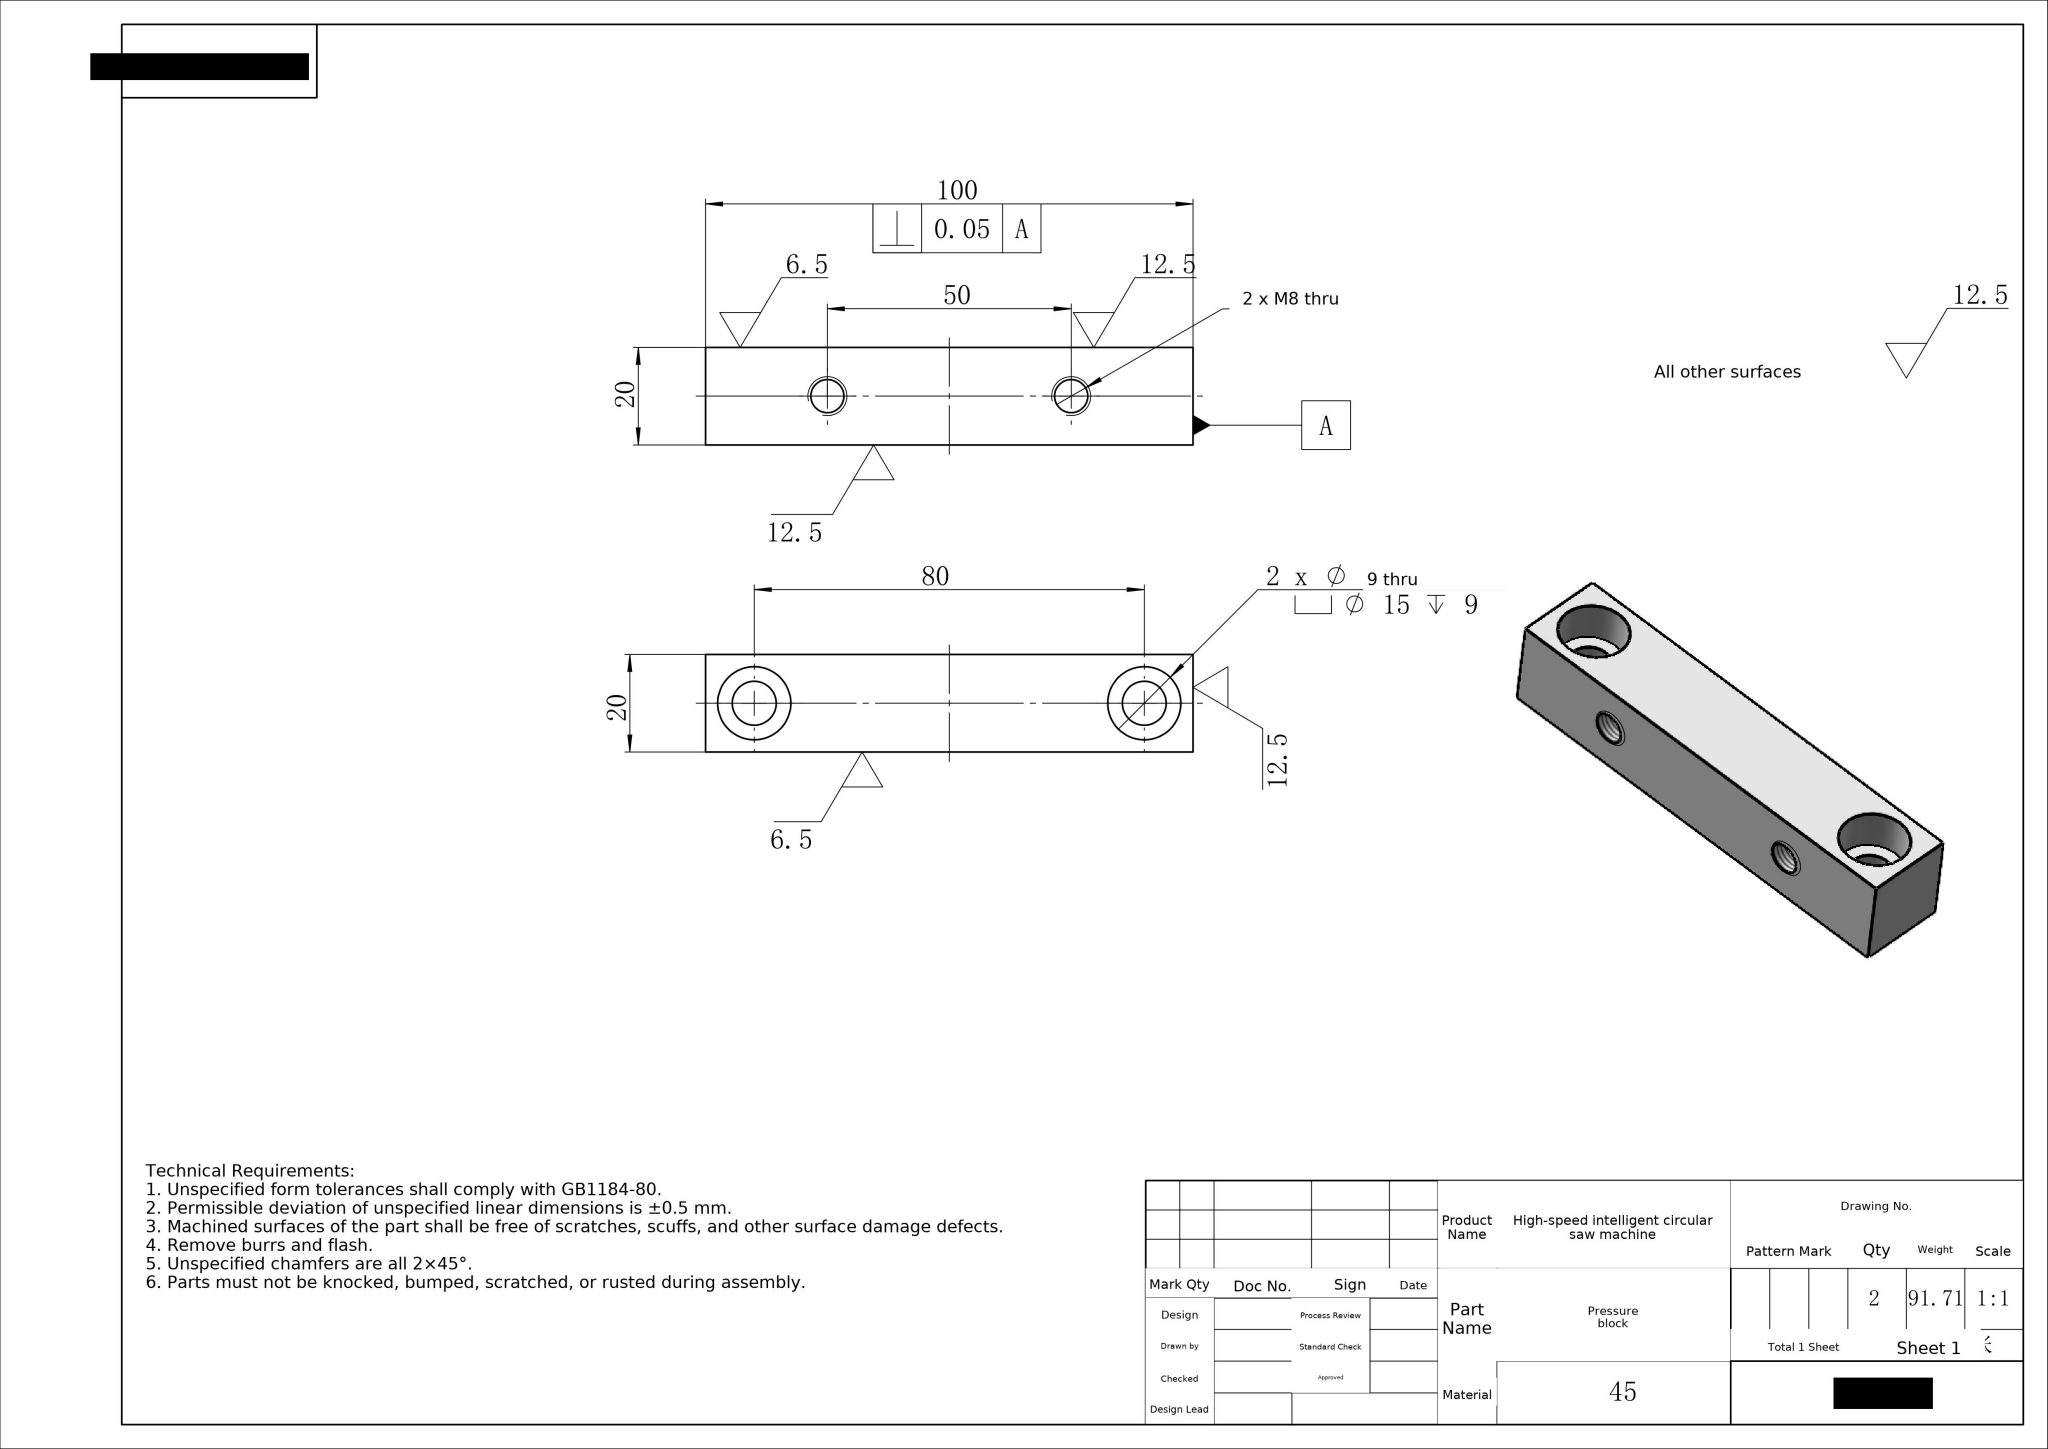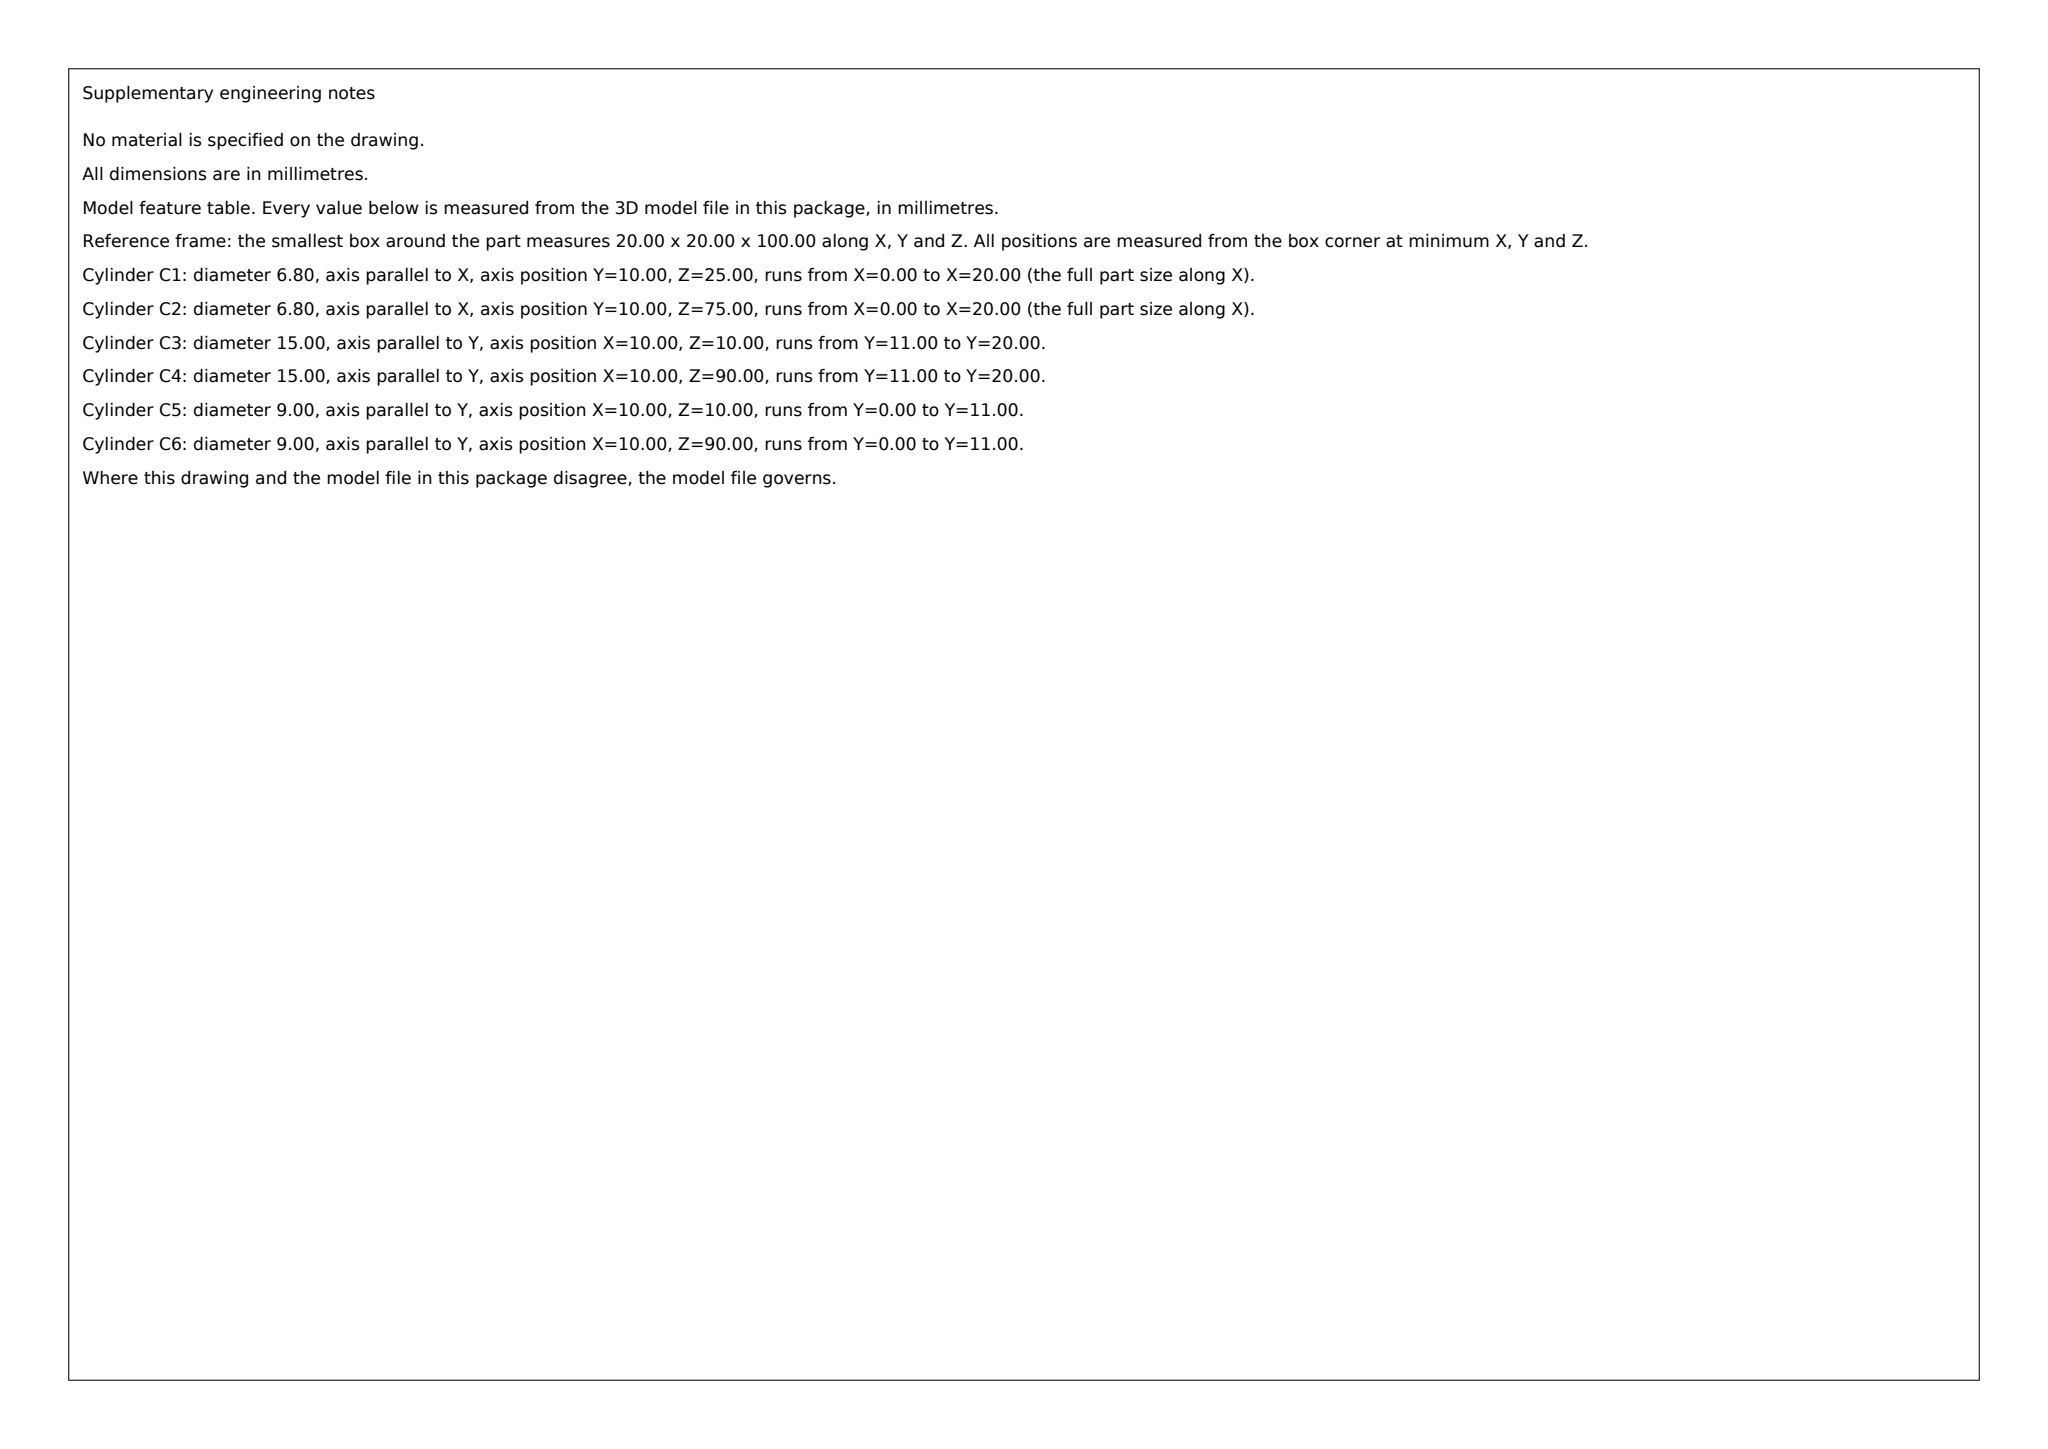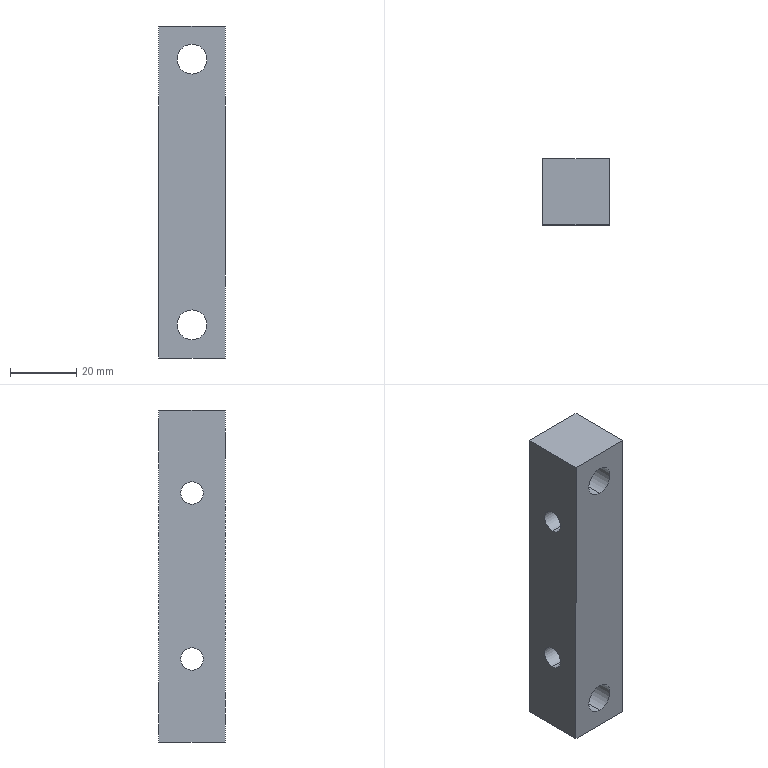Part | SolidWorks | mm | 1 solid | 20 faces | box 20 x 20 x 100 mm | volume 33967 mm3 | cylinder 12 | plane 8 | commonest cylinder face diameters 6.8 x4 15 x4 9 x4
build123d program:
from build123d import *

# Parameters (mm, degrees)
SKETCH2_W                                            = 20
SKETCH2_H                                            = 100
BOSS_EXTRUDE1_DEPTH                                  = 20
HOLE_SIZE_ACCORDING_TO_HEXAGON_SOCKET_HE_D           = 9
HOLE_SIZE_ACCORDING_TO_HEXAGON_SOCKET_HE_CBORE_D     = 15
HOLE_SIZE_ACCORDING_TO_HEXAGON_SOCKET_HE_CBORE_DEPTH = 9
M8_TAPPED_HOLE1_D                                    = 6.8


with BuildPart() as part:
    # Sketch2 → Boss-Extrude1 (new body)
    with BuildSketch(Plane(origin=(0, 0, 0), x_dir=(1, 0, 0), z_dir=(0, 1, 0))):
        Rectangle(SKETCH2_W, SKETCH2_H)
    extrude(amount=BOSS_EXTRUDE1_DEPTH)

    # Hole Size_According to_Hexagon Socket He (through all)
    with Locations(Plane(origin=(0, 20, -40), x_dir=(0, 0, 1), z_dir=(0, 1, 0))):
        with Locations((0, 0), (80, 0)):
            CounterBoreHole(HOLE_SIZE_ACCORDING_TO_HEXAGON_SOCKET_HE_D / 2, HOLE_SIZE_ACCORDING_TO_HEXAGON_SOCKET_HE_CBORE_D / 2, HOLE_SIZE_ACCORDING_TO_HEXAGON_SOCKET_HE_CBORE_DEPTH)

    # M8 Tapped Hole1 (through all)
    with Locations(Plane(origin=(-10, 10, -25), x_dir=(0, 0, -1), z_dir=(-1, 0, 0))):
        with Locations((0, 0), (-50, 0)):
            Hole(M8_TAPPED_HOLE1_D / 2)


solid = part.part
STEP:
#1=CARTESIAN_POINT('',(10.,10.,-28.4));
#2=VERTEX_POINT('',#1);
#3=CARTESIAN_POINT('',(10.,10.,-21.6));
#4=VERTEX_POINT('',#3);
#5=CARTESIAN_POINT('',(10.,10.,-25.));
#6=DIRECTION('',(-1.,0.,0.));
#7=DIRECTION('',(0.,0.,1.));
#8=AXIS2_PLACEMENT_3D('',#5,#6,#7);
#9=CIRCLE('',#8,3.4);
#10=EDGE_CURVE('',#2,#4,#9,.T.);
#11=ORIENTED_EDGE('',*,*,#10,.F.);
#12=CARTESIAN_POINT('',(-10.,10.,-28.4));
#13=VERTEX_POINT('',#12);
#14=CARTESIAN_POINT('',(-10.,10.,-28.4));
#15=DIRECTION('',(-1.,0.,0.));
#16=VECTOR('',#15,1000.);
#17=LINE('',#14,#16);
#18=EDGE_CURVE('',#2,#13,#17,.T.);
#19=ORIENTED_EDGE('',*,*,#18,.T.);
#20=CARTESIAN_POINT('',(-10.,10.,-21.6));
#21=VERTEX_POINT('',#20);
#22=CARTESIAN_POINT('',(-10.,10.,-25.));
#23=DIRECTION('',(-1.,0.,0.));
#24=DIRECTION('',(0.,0.,1.));
#25=AXIS2_PLACEMENT_3D('',#22,#23,#24);
#26=CIRCLE('',#25,3.4);
#27=EDGE_CURVE('',#13,#21,#26,.T.);
#28=ORIENTED_EDGE('',*,*,#27,.T.);
#29=CARTESIAN_POINT('',(-10.,10.,-21.6));
#30=DIRECTION('',(-1.,0.,0.));
#31=VECTOR('',#30,1000.);
#32=LINE('',#29,#31);
#33=EDGE_CURVE('',#4,#21,#32,.T.);
#34=ORIENTED_EDGE('',*,*,#33,.F.);
#35=EDGE_LOOP('',(#11,#19,#28,#34));
#36=FACE_OUTER_BOUND('',#35,.T.);
#37=CARTESIAN_POINT('',(-10.,10.,-25.));
#38=DIRECTION('',(-1.,0.,0.));
#39=DIRECTION('',(0.,0.,1.));
#40=AXIS2_PLACEMENT_3D('',#37,#38,#39);
#41=CYLINDRICAL_SURFACE('',#40,3.4);
#42=ADVANCED_FACE('',(#36),#41,.F.);
#43=CARTESIAN_POINT('',(10.,10.,21.6));
#44=VERTEX_POINT('',#43);
#45=CARTESIAN_POINT('',(10.,10.,28.4));
#46=VERTEX_POINT('',#45);
#47=CARTESIAN_POINT('',(10.,10.,25.));
#48=DIRECTION('',(-1.,0.,0.));
#49=DIRECTION('',(0.,0.,1.));
#50=AXIS2_PLACEMENT_3D('',#47,#48,#49);
#51=CIRCLE('',#50,3.4);
#52=EDGE_CURVE('',#44,#46,#51,.T.);
#53=ORIENTED_EDGE('',*,*,#52,.F.);
#54=CARTESIAN_POINT('',(-10.,10.,21.6));
#55=VERTEX_POINT('',#54);
#56=CARTESIAN_POINT('',(-10.,10.,21.6));
#57=DIRECTION('',(-1.,0.,0.));
#58=VECTOR('',#57,1000.);
#59=LINE('',#56,#58);
#60=EDGE_CURVE('',#44,#55,#59,.T.);
#61=ORIENTED_EDGE('',*,*,#60,.T.);
#62=CARTESIAN_POINT('',(-10.,10.,28.4));
#63=VERTEX_POINT('',#62);
#64=CARTESIAN_POINT('',(-10.,10.,25.));
#65=DIRECTION('',(-1.,0.,0.));
#66=DIRECTION('',(0.,0.,1.));
#67=AXIS2_PLACEMENT_3D('',#64,#65,#66);
#68=CIRCLE('',#67,3.4);
#69=EDGE_CURVE('',#55,#63,#68,.T.);
#70=ORIENTED_EDGE('',*,*,#69,.T.);
#71=CARTESIAN_POINT('',(-10.,10.,28.4));
#72=DIRECTION('',(-1.,0.,0.));
#73=VECTOR('',#72,1000.);
#74=LINE('',#71,#73);
#75=EDGE_CURVE('',#46,#63,#74,.T.);
#76=ORIENTED_EDGE('',*,*,#75,.F.);
#77=EDGE_LOOP('',(#53,#61,#70,#76));
#78=FACE_OUTER_BOUND('',#77,.T.);
#79=CARTESIAN_POINT('',(-10.,10.,25.));
#80=DIRECTION('',(-1.,0.,0.));
#81=DIRECTION('',(0.,0.,1.));
#82=AXIS2_PLACEMENT_3D('',#79,#80,#81);
#83=CYLINDRICAL_SURFACE('',#82,3.4);
#84=ADVANCED_FACE('',(#78),#83,.F.);
#85=CARTESIAN_POINT('',(0.,11.,-47.5));
#86=VERTEX_POINT('',#85);
#87=CARTESIAN_POINT('',(0.,11.,-32.5));
#88=VERTEX_POINT('',#87);
#89=CARTESIAN_POINT('',(0.,11.,-40.));
#90=DIRECTION('',(0.,1.,0.));
#91=DIRECTION('',(0.,0.,1.));
#92=AXIS2_PLACEMENT_3D('',#89,#90,#91);
#93=CIRCLE('',#92,7.5);
#94=EDGE_CURVE('',#86,#88,#93,.T.);
#95=ORIENTED_EDGE('',*,*,#94,.F.);
#96=CARTESIAN_POINT('',(0.,20.,-47.5));
#97=VERTEX_POINT('',#96);
#98=CARTESIAN_POINT('',(0.,20.,-47.5));
#99=DIRECTION('',(0.,1.,0.));
#100=VECTOR('',#99,1000.);
#101=LINE('',#98,#100);
#102=EDGE_CURVE('',#86,#97,#101,.T.);
#103=ORIENTED_EDGE('',*,*,#102,.T.);
#104=CARTESIAN_POINT('',(0.,20.,-32.5));
#105=VERTEX_POINT('',#104);
#106=CARTESIAN_POINT('',(0.,20.,-40.));
#107=DIRECTION('',(0.,1.,0.));
#108=DIRECTION('',(0.,0.,1.));
#109=AXIS2_PLACEMENT_3D('',#106,#107,#108);
#110=CIRCLE('',#109,7.5);
#111=EDGE_CURVE('',#97,#105,#110,.T.);
#112=ORIENTED_EDGE('',*,*,#111,.T.);
#113=CARTESIAN_POINT('',(0.,20.,-32.5));
#114=DIRECTION('',(0.,1.,0.));
#115=VECTOR('',#114,1000.);
#116=LINE('',#113,#115);
#117=EDGE_CURVE('',#88,#105,#116,.T.);
#118=ORIENTED_EDGE('',*,*,#117,.F.);
#119=EDGE_LOOP('',(#95,#103,#112,#118));
#120=FACE_OUTER_BOUND('',#119,.T.);
#121=CARTESIAN_POINT('',(0.,20.,-40.));
#122=DIRECTION('',(0.,1.,0.));
#123=DIRECTION('',(0.,0.,1.));
#124=AXIS2_PLACEMENT_3D('',#121,#122,#123);
#125=CYLINDRICAL_SURFACE('',#124,7.5);
#126=ADVANCED_FACE('',(#120),#125,.F.);
#127=CARTESIAN_POINT('',(0.,0.,-44.5));
#128=VERTEX_POINT('',#127);
#129=CARTESIAN_POINT('',(0.,0.,-35.5));
#130=VERTEX_POINT('',#129);
#131=CARTESIAN_POINT('',(0.,0.,-40.));
#132=DIRECTION('',(0.,1.,0.));
#133=DIRECTION('',(0.,0.,1.));
#134=AXIS2_PLACEMENT_3D('',#131,#132,#133);
#135=CIRCLE('',#134,4.5);
#136=EDGE_CURVE('',#128,#130,#135,.T.);
#137=ORIENTED_EDGE('',*,*,#136,.F.);
#138=CARTESIAN_POINT('',(0.,11.,-44.5));
#139=VERTEX_POINT('',#138);
#140=CARTESIAN_POINT('',(0.,20.,-44.5));
#141=DIRECTION('',(0.,1.,0.));
#142=VECTOR('',#141,1000.);
#143=LINE('',#140,#142);
#144=EDGE_CURVE('',#128,#139,#143,.T.);
#145=ORIENTED_EDGE('',*,*,#144,.T.);
#146=CARTESIAN_POINT('',(0.,11.,-35.5));
#147=VERTEX_POINT('',#146);
#148=CARTESIAN_POINT('',(0.,11.,-40.));
#149=DIRECTION('',(0.,1.,0.));
#150=DIRECTION('',(0.,0.,1.));
#151=AXIS2_PLACEMENT_3D('',#148,#149,#150);
#152=CIRCLE('',#151,4.5);
#153=EDGE_CURVE('',#139,#147,#152,.T.);
#154=ORIENTED_EDGE('',*,*,#153,.T.);
#155=CARTESIAN_POINT('',(0.,20.,-35.5));
#156=DIRECTION('',(0.,1.,0.));
#157=VECTOR('',#156,1000.);
#158=LINE('',#155,#157);
#159=EDGE_CURVE('',#130,#147,#158,.T.);
#160=ORIENTED_EDGE('',*,*,#159,.F.);
#161=EDGE_LOOP('',(#137,#145,#154,#160));
#162=FACE_OUTER_BOUND('',#161,.T.);
#163=CARTESIAN_POINT('',(0.,20.,-40.));
#164=DIRECTION('',(0.,1.,0.));
#165=DIRECTION('',(0.,0.,1.));
#166=AXIS2_PLACEMENT_3D('',#163,#164,#165);
#167=CYLINDRICAL_SURFACE('',#166,4.5);
#168=ADVANCED_FACE('',(#162),#167,.F.);
#169=CARTESIAN_POINT('',(0.,11.,32.5));
#170=VERTEX_POINT('',#169);
#171=CARTESIAN_POINT('',(0.,11.,47.5));
#172=VERTEX_POINT('',#171);
#173=CARTESIAN_POINT('',(0.,11.,40.));
#174=DIRECTION('',(0.,1.,0.));
#175=DIRECTION('',(0.,0.,1.));
#176=AXIS2_PLACEMENT_3D('',#173,#174,#175);
#177=CIRCLE('',#176,7.5);
#178=EDGE_CURVE('',#170,#172,#177,.T.);
#179=ORIENTED_EDGE('',*,*,#178,.F.);
#180=CARTESIAN_POINT('',(0.,20.,32.5));
#181=VERTEX_POINT('',#180);
#182=CARTESIAN_POINT('',(0.,20.,32.5));
#183=DIRECTION('',(0.,1.,0.));
#184=VECTOR('',#183,1000.);
#185=LINE('',#182,#184);
#186=EDGE_CURVE('',#170,#181,#185,.T.);
#187=ORIENTED_EDGE('',*,*,#186,.T.);
#188=CARTESIAN_POINT('',(0.,20.,47.5));
#189=VERTEX_POINT('',#188);
#190=CARTESIAN_POINT('',(0.,20.,40.));
#191=DIRECTION('',(0.,1.,0.));
#192=DIRECTION('',(0.,0.,1.));
#193=AXIS2_PLACEMENT_3D('',#190,#191,#192);
#194=CIRCLE('',#193,7.5);
#195=EDGE_CURVE('',#181,#189,#194,.T.);
#196=ORIENTED_EDGE('',*,*,#195,.T.);
#197=CARTESIAN_POINT('',(0.,20.,47.5));
#198=DIRECTION('',(0.,1.,0.));
#199=VECTOR('',#198,1000.);
#200=LINE('',#197,#199);
#201=EDGE_CURVE('',#172,#189,#200,.T.);
#202=ORIENTED_EDGE('',*,*,#201,.F.);
#203=EDGE_LOOP('',(#179,#187,#196,#202));
#204=FACE_OUTER_BOUND('',#203,.T.);
#205=CARTESIAN_POINT('',(0.,20.,40.));
#206=DIRECTION('',(0.,1.,0.));
#207=DIRECTION('',(0.,0.,1.));
#208=AXIS2_PLACEMENT_3D('',#205,#206,#207);
#209=CYLINDRICAL_SURFACE('',#208,7.5);
#210=ADVANCED_FACE('',(#204),#209,.F.);
#211=CARTESIAN_POINT('',(0.,0.,35.5));
#212=VERTEX_POINT('',#211);
#213=CARTESIAN_POINT('',(0.,0.,44.5));
#214=VERTEX_POINT('',#213);
#215=CARTESIAN_POINT('',(0.,0.,40.));
#216=DIRECTION('',(0.,1.,0.));
#217=DIRECTION('',(0.,0.,1.));
#218=AXIS2_PLACEMENT_3D('',#215,#216,#217);
#219=CIRCLE('',#218,4.5);
#220=EDGE_CURVE('',#212,#214,#219,.T.);
#221=ORIENTED_EDGE('',*,*,#220,.F.);
#222=CARTESIAN_POINT('',(0.,11.,35.5));
#223=VERTEX_POINT('',#222);
#224=CARTESIAN_POINT('',(0.,20.,35.5));
#225=DIRECTION('',(0.,1.,0.));
#226=VECTOR('',#225,1000.);
#227=LINE('',#224,#226);
#228=EDGE_CURVE('',#212,#223,#227,.T.);
#229=ORIENTED_EDGE('',*,*,#228,.T.);
#230=CARTESIAN_POINT('',(0.,11.,44.5));
#231=VERTEX_POINT('',#230);
#232=CARTESIAN_POINT('',(0.,11.,40.));
#233=DIRECTION('',(0.,1.,0.));
#234=DIRECTION('',(0.,0.,1.));
#235=AXIS2_PLACEMENT_3D('',#232,#233,#234);
#236=CIRCLE('',#235,4.5);
#237=EDGE_CURVE('',#223,#231,#236,.T.);
#238=ORIENTED_EDGE('',*,*,#237,.T.);
#239=CARTESIAN_POINT('',(0.,20.,44.5));
#240=DIRECTION('',(0.,1.,0.));
#241=VECTOR('',#240,1000.);
#242=LINE('',#239,#241);
#243=EDGE_CURVE('',#214,#231,#242,.T.);
#244=ORIENTED_EDGE('',*,*,#243,.F.);
#245=EDGE_LOOP('',(#221,#229,#238,#244));
#246=FACE_OUTER_BOUND('',#245,.T.);
#247=CARTESIAN_POINT('',(0.,20.,40.));
#248=DIRECTION('',(0.,1.,0.));
#249=DIRECTION('',(0.,0.,1.));
#250=AXIS2_PLACEMENT_3D('',#247,#248,#249);
#251=CYLINDRICAL_SURFACE('',#250,4.5);
#252=ADVANCED_FACE('',(#246),#251,.F.);
#253=CARTESIAN_POINT('',(10.,10.,-25.));
#254=DIRECTION('',(-1.,0.,0.));
#255=DIRECTION('',(0.,0.,1.));
#256=AXIS2_PLACEMENT_3D('',#253,#254,#255);
#257=CIRCLE('',#256,3.4);
#258=EDGE_CURVE('',#4,#2,#257,.T.);
#259=ORIENTED_EDGE('',*,*,#258,.T.);
#260=ORIENTED_EDGE('',*,*,#10,.T.);
#261=EDGE_LOOP('',(#259,#260));
#262=FACE_BOUND('',#261,.T.);
#263=CARTESIAN_POINT('',(10.,10.,25.));
#264=DIRECTION('',(-1.,0.,0.));
#265=DIRECTION('',(0.,0.,1.));
#266=AXIS2_PLACEMENT_3D('',#263,#264,#265);
#267=CIRCLE('',#266,3.4);
#268=EDGE_CURVE('',#46,#44,#267,.T.);
#269=ORIENTED_EDGE('',*,*,#268,.T.);
#270=ORIENTED_EDGE('',*,*,#52,.T.);
#271=EDGE_LOOP('',(#269,#270));
#272=FACE_BOUND('',#271,.T.);
#273=CARTESIAN_POINT('',(10.,0.,50.));
#274=VERTEX_POINT('',#273);
#275=CARTESIAN_POINT('',(10.,0.,-50.));
#276=VERTEX_POINT('',#275);
#277=CARTESIAN_POINT('',(10.,0.,-50.));
#278=DIRECTION('',(-0.,0.,-1.));
#279=VECTOR('',#278,1000.);
#280=LINE('',#277,#279);
#281=EDGE_CURVE('',#274,#276,#280,.T.);
#282=ORIENTED_EDGE('',*,*,#281,.T.);
#283=CARTESIAN_POINT('',(10.,20.,-50.));
#284=VERTEX_POINT('',#283);
#285=CARTESIAN_POINT('',(10.,20.,-50.));
#286=DIRECTION('',(0.,-1.,0.));
#287=VECTOR('',#286,1000.);
#288=LINE('',#285,#287);
#289=EDGE_CURVE('',#284,#276,#288,.T.);
#290=ORIENTED_EDGE('',*,*,#289,.F.);
#291=CARTESIAN_POINT('',(10.,20.,50.));
#292=VERTEX_POINT('',#291);
#293=CARTESIAN_POINT('',(10.,20.,-50.));
#294=DIRECTION('',(-0.,0.,-1.));
#295=VECTOR('',#294,1000.);
#296=LINE('',#293,#295);
#297=EDGE_CURVE('',#292,#284,#296,.T.);
#298=ORIENTED_EDGE('',*,*,#297,.F.);
#299=CARTESIAN_POINT('',(10.,20.,50.));
#300=DIRECTION('',(0.,-1.,0.));
#301=VECTOR('',#300,1000.);
#302=LINE('',#299,#301);
#303=EDGE_CURVE('',#292,#274,#302,.T.);
#304=ORIENTED_EDGE('',*,*,#303,.T.);
#305=EDGE_LOOP('',(#282,#290,#298,#304));
#306=FACE_OUTER_BOUND('',#305,.T.);
#307=CARTESIAN_POINT('',(10.,20.,-50.));
#308=DIRECTION('',(-1.,0.,0.));
#309=DIRECTION('',(0.,0.,1.));
#310=AXIS2_PLACEMENT_3D('',#307,#308,#309);
#311=PLANE('',#310);
#312=ADVANCED_FACE('',(#262,#272,#306),#311,.F.);
#313=CARTESIAN_POINT('',(-10.,0.,-50.));
#314=VERTEX_POINT('',#313);
#315=CARTESIAN_POINT('',(-10.,0.,-50.));
#316=DIRECTION('',(-1.,0.,0.));
#317=VECTOR('',#316,1000.);
#318=LINE('',#315,#317);
#319=EDGE_CURVE('',#276,#314,#318,.T.);
#320=ORIENTED_EDGE('',*,*,#319,.T.);
#321=CARTESIAN_POINT('',(-10.,20.,-50.));
#322=VERTEX_POINT('',#321);
#323=CARTESIAN_POINT('',(-10.,20.,-50.));
#324=DIRECTION('',(0.,-1.,0.));
#325=VECTOR('',#324,1000.);
#326=LINE('',#323,#325);
#327=EDGE_CURVE('',#322,#314,#326,.T.);
#328=ORIENTED_EDGE('',*,*,#327,.F.);
#329=CARTESIAN_POINT('',(-10.,20.,-50.));
#330=DIRECTION('',(-1.,0.,0.));
#331=VECTOR('',#330,1000.);
#332=LINE('',#329,#331);
#333=EDGE_CURVE('',#284,#322,#332,.T.);
#334=ORIENTED_EDGE('',*,*,#333,.F.);
#335=ORIENTED_EDGE('',*,*,#289,.T.);
#336=EDGE_LOOP('',(#320,#328,#334,#335));
#337=FACE_OUTER_BOUND('',#336,.T.);
#338=CARTESIAN_POINT('',(-10.,20.,-50.));
#339=DIRECTION('',(0.,0.,1.));
#340=DIRECTION('',(1.,0.,0.));
#341=AXIS2_PLACEMENT_3D('',#338,#339,#340);
#342=PLANE('',#341);
#343=ADVANCED_FACE('',(#337),#342,.F.);
#344=CARTESIAN_POINT('',(-10.,10.,-25.));
#345=DIRECTION('',(-1.,0.,0.));
#346=DIRECTION('',(0.,0.,1.));
#347=AXIS2_PLACEMENT_3D('',#344,#345,#346);
#348=CIRCLE('',#347,3.4);
#349=EDGE_CURVE('',#21,#13,#348,.T.);
#350=ORIENTED_EDGE('',*,*,#349,.F.);
#351=ORIENTED_EDGE('',*,*,#27,.F.);
#352=EDGE_LOOP('',(#350,#351));
#353=FACE_BOUND('',#352,.T.);
#354=CARTESIAN_POINT('',(-10.,10.,25.));
#355=DIRECTION('',(-1.,0.,0.));
#356=DIRECTION('',(0.,0.,1.));
#357=AXIS2_PLACEMENT_3D('',#354,#355,#356);
#358=CIRCLE('',#357,3.4);
#359=EDGE_CURVE('',#63,#55,#358,.T.);
#360=ORIENTED_EDGE('',*,*,#359,.F.);
#361=ORIENTED_EDGE('',*,*,#69,.F.);
#362=EDGE_LOOP('',(#360,#361));
#363=FACE_BOUND('',#362,.T.);
#364=CARTESIAN_POINT('',(-10.,0.,50.));
#365=VERTEX_POINT('',#364);
#366=CARTESIAN_POINT('',(-10.,0.,-50.));
#367=DIRECTION('',(0.,0.,1.));
#368=VECTOR('',#367,1000.);
#369=LINE('',#366,#368);
#370=EDGE_CURVE('',#314,#365,#369,.T.);
#371=ORIENTED_EDGE('',*,*,#370,.T.);
#372=CARTESIAN_POINT('',(-10.,20.,50.));
#373=VERTEX_POINT('',#372);
#374=CARTESIAN_POINT('',(-10.,20.,50.));
#375=DIRECTION('',(0.,-1.,0.));
#376=VECTOR('',#375,1000.);
#377=LINE('',#374,#376);
#378=EDGE_CURVE('',#373,#365,#377,.T.);
#379=ORIENTED_EDGE('',*,*,#378,.F.);
#380=CARTESIAN_POINT('',(-10.,20.,-50.));
#381=DIRECTION('',(0.,0.,1.));
#382=VECTOR('',#381,1000.);
#383=LINE('',#380,#382);
#384=EDGE_CURVE('',#322,#373,#383,.T.);
#385=ORIENTED_EDGE('',*,*,#384,.F.);
#386=ORIENTED_EDGE('',*,*,#327,.T.);
#387=EDGE_LOOP('',(#371,#379,#385,#386));
#388=FACE_OUTER_BOUND('',#387,.T.);
#389=CARTESIAN_POINT('',(-10.,20.,-50.));
#390=DIRECTION('',(1.,0.,-0.));
#391=DIRECTION('',(-0.,0.,-1.));
#392=AXIS2_PLACEMENT_3D('',#389,#390,#391);
#393=PLANE('',#392);
#394=ADVANCED_FACE('',(#353,#363,#388),#393,.F.);
#395=CARTESIAN_POINT('',(-10.,0.,50.));
#396=DIRECTION('',(1.,0.,0.));
#397=VECTOR('',#396,1000.);
#398=LINE('',#395,#397);
#399=EDGE_CURVE('',#365,#274,#398,.T.);
#400=ORIENTED_EDGE('',*,*,#399,.T.);
#401=ORIENTED_EDGE('',*,*,#303,.F.);
#402=CARTESIAN_POINT('',(-10.,20.,50.));
#403=DIRECTION('',(1.,0.,0.));
#404=VECTOR('',#403,1000.);
#405=LINE('',#402,#404);
#406=EDGE_CURVE('',#373,#292,#405,.T.);
#407=ORIENTED_EDGE('',*,*,#406,.F.);
#408=ORIENTED_EDGE('',*,*,#378,.T.);
#409=EDGE_LOOP('',(#400,#401,#407,#408));
#410=FACE_OUTER_BOUND('',#409,.T.);
#411=CARTESIAN_POINT('',(-10.,20.,50.));
#412=DIRECTION('',(0.,0.,-1.));
#413=DIRECTION('',(-1.,0.,0.));
#414=AXIS2_PLACEMENT_3D('',#411,#412,#413);
#415=PLANE('',#414);
#416=ADVANCED_FACE('',(#410),#415,.F.);
#417=CARTESIAN_POINT('',(0.,20.,-40.));
#418=DIRECTION('',(0.,1.,0.));
#419=DIRECTION('',(0.,0.,1.));
#420=AXIS2_PLACEMENT_3D('',#417,#418,#419);
#421=CIRCLE('',#420,7.5);
#422=EDGE_CURVE('',#105,#97,#421,.T.);
#423=ORIENTED_EDGE('',*,*,#422,.F.);
#424=ORIENTED_EDGE('',*,*,#111,.F.);
#425=EDGE_LOOP('',(#423,#424));
#426=FACE_BOUND('',#425,.T.);
#427=CARTESIAN_POINT('',(0.,20.,40.));
#428=DIRECTION('',(0.,1.,0.));
#429=DIRECTION('',(0.,0.,1.));
#430=AXIS2_PLACEMENT_3D('',#427,#428,#429);
#431=CIRCLE('',#430,7.5);
#432=EDGE_CURVE('',#189,#181,#431,.T.);
#433=ORIENTED_EDGE('',*,*,#432,.F.);
#434=ORIENTED_EDGE('',*,*,#195,.F.);
#435=EDGE_LOOP('',(#433,#434));
#436=FACE_BOUND('',#435,.T.);
#437=ORIENTED_EDGE('',*,*,#297,.T.);
#438=ORIENTED_EDGE('',*,*,#333,.T.);
#439=ORIENTED_EDGE('',*,*,#384,.T.);
#440=ORIENTED_EDGE('',*,*,#406,.T.);
#441=EDGE_LOOP('',(#437,#438,#439,#440));
#442=FACE_OUTER_BOUND('',#441,.T.);
#443=CARTESIAN_POINT('',(0.,20.,0.));
#444=DIRECTION('',(0.,1.,0.));
#445=DIRECTION('',(0.,0.,1.));
#446=AXIS2_PLACEMENT_3D('',#443,#444,#445);
#447=PLANE('',#446);
#448=ADVANCED_FACE('',(#426,#436,#442),#447,.T.);
#449=CARTESIAN_POINT('',(0.,0.,-40.));
#450=DIRECTION('',(0.,1.,0.));
#451=DIRECTION('',(0.,0.,1.));
#452=AXIS2_PLACEMENT_3D('',#449,#450,#451);
#453=CIRCLE('',#452,4.5);
#454=EDGE_CURVE('',#130,#128,#453,.T.);
#455=ORIENTED_EDGE('',*,*,#454,.T.);
#456=ORIENTED_EDGE('',*,*,#136,.T.);
#457=EDGE_LOOP('',(#455,#456));
#458=FACE_BOUND('',#457,.T.);
#459=CARTESIAN_POINT('',(0.,0.,40.));
#460=DIRECTION('',(0.,1.,0.));
#461=DIRECTION('',(0.,0.,1.));
#462=AXIS2_PLACEMENT_3D('',#459,#460,#461);
#463=CIRCLE('',#462,4.5);
#464=EDGE_CURVE('',#214,#212,#463,.T.);
#465=ORIENTED_EDGE('',*,*,#464,.T.);
#466=ORIENTED_EDGE('',*,*,#220,.T.);
#467=EDGE_LOOP('',(#465,#466));
#468=FACE_BOUND('',#467,.T.);
#469=ORIENTED_EDGE('',*,*,#281,.F.);
#470=ORIENTED_EDGE('',*,*,#399,.F.);
#471=ORIENTED_EDGE('',*,*,#370,.F.);
#472=ORIENTED_EDGE('',*,*,#319,.F.);
#473=EDGE_LOOP('',(#469,#470,#471,#472));
#474=FACE_OUTER_BOUND('',#473,.T.);
#475=CARTESIAN_POINT('',(0.,0.,0.));
#476=DIRECTION('',(0.,1.,0.));
#477=DIRECTION('',(0.,0.,1.));
#478=AXIS2_PLACEMENT_3D('',#475,#476,#477);
#479=PLANE('',#478);
#480=ADVANCED_FACE('',(#458,#468,#474),#479,.F.);
#481=ORIENTED_EDGE('',*,*,#228,.F.);
#482=ORIENTED_EDGE('',*,*,#464,.F.);
#483=ORIENTED_EDGE('',*,*,#243,.T.);
#484=CARTESIAN_POINT('',(0.,11.,40.));
#485=DIRECTION('',(0.,1.,0.));
#486=DIRECTION('',(0.,0.,1.));
#487=AXIS2_PLACEMENT_3D('',#484,#485,#486);
#488=CIRCLE('',#487,4.5);
#489=EDGE_CURVE('',#231,#223,#488,.T.);
#490=ORIENTED_EDGE('',*,*,#489,.T.);
#491=EDGE_LOOP('',(#481,#482,#483,#490));
#492=FACE_OUTER_BOUND('',#491,.T.);
#493=CARTESIAN_POINT('',(0.,20.,40.));
#494=DIRECTION('',(0.,1.,0.));
#495=DIRECTION('',(0.,0.,1.));
#496=AXIS2_PLACEMENT_3D('',#493,#494,#495);
#497=CYLINDRICAL_SURFACE('',#496,4.5);
#498=ADVANCED_FACE('',(#492),#497,.F.);
#499=ORIENTED_EDGE('',*,*,#489,.F.);
#500=ORIENTED_EDGE('',*,*,#237,.F.);
#501=EDGE_LOOP('',(#499,#500));
#502=FACE_BOUND('',#501,.T.);
#503=CARTESIAN_POINT('',(0.,11.,40.));
#504=DIRECTION('',(0.,1.,0.));
#505=DIRECTION('',(0.,0.,1.));
#506=AXIS2_PLACEMENT_3D('',#503,#504,#505);
#507=CIRCLE('',#506,7.5);
#508=EDGE_CURVE('',#172,#170,#507,.T.);
#509=ORIENTED_EDGE('',*,*,#508,.T.);
#510=ORIENTED_EDGE('',*,*,#178,.T.);
#511=EDGE_LOOP('',(#509,#510));
#512=FACE_OUTER_BOUND('',#511,.T.);
#513=CARTESIAN_POINT('',(4.5,11.,40.));
#514=DIRECTION('',(0.,-1.,0.));
#515=DIRECTION('',(0.,0.,-1.));
#516=AXIS2_PLACEMENT_3D('',#513,#514,#515);
#517=PLANE('',#516);
#518=ADVANCED_FACE('',(#502,#512),#517,.F.);
#519=ORIENTED_EDGE('',*,*,#186,.F.);
#520=ORIENTED_EDGE('',*,*,#508,.F.);
#521=ORIENTED_EDGE('',*,*,#201,.T.);
#522=ORIENTED_EDGE('',*,*,#432,.T.);
#523=EDGE_LOOP('',(#519,#520,#521,#522));
#524=FACE_OUTER_BOUND('',#523,.T.);
#525=CARTESIAN_POINT('',(0.,20.,40.));
#526=DIRECTION('',(0.,1.,0.));
#527=DIRECTION('',(0.,0.,1.));
#528=AXIS2_PLACEMENT_3D('',#525,#526,#527);
#529=CYLINDRICAL_SURFACE('',#528,7.5);
#530=ADVANCED_FACE('',(#524),#529,.F.);
#531=ORIENTED_EDGE('',*,*,#144,.F.);
#532=ORIENTED_EDGE('',*,*,#454,.F.);
#533=ORIENTED_EDGE('',*,*,#159,.T.);
#534=CARTESIAN_POINT('',(0.,11.,-40.));
#535=DIRECTION('',(0.,1.,0.));
#536=DIRECTION('',(0.,0.,1.));
#537=AXIS2_PLACEMENT_3D('',#534,#535,#536);
#538=CIRCLE('',#537,4.5);
#539=EDGE_CURVE('',#147,#139,#538,.T.);
#540=ORIENTED_EDGE('',*,*,#539,.T.);
#541=EDGE_LOOP('',(#531,#532,#533,#540));
#542=FACE_OUTER_BOUND('',#541,.T.);
#543=CARTESIAN_POINT('',(0.,20.,-40.));
#544=DIRECTION('',(0.,1.,0.));
#545=DIRECTION('',(0.,0.,1.));
#546=AXIS2_PLACEMENT_3D('',#543,#544,#545);
#547=CYLINDRICAL_SURFACE('',#546,4.5);
#548=ADVANCED_FACE('',(#542),#547,.F.);
#549=ORIENTED_EDGE('',*,*,#539,.F.);
#550=ORIENTED_EDGE('',*,*,#153,.F.);
#551=EDGE_LOOP('',(#549,#550));
#552=FACE_BOUND('',#551,.T.);
#553=CARTESIAN_POINT('',(0.,11.,-40.));
#554=DIRECTION('',(0.,1.,0.));
#555=DIRECTION('',(0.,0.,1.));
#556=AXIS2_PLACEMENT_3D('',#553,#554,#555);
#557=CIRCLE('',#556,7.5);
#558=EDGE_CURVE('',#88,#86,#557,.T.);
#559=ORIENTED_EDGE('',*,*,#558,.T.);
#560=ORIENTED_EDGE('',*,*,#94,.T.);
#561=EDGE_LOOP('',(#559,#560));
#562=FACE_OUTER_BOUND('',#561,.T.);
#563=CARTESIAN_POINT('',(4.5,11.,-40.));
#564=DIRECTION('',(0.,-1.,0.));
#565=DIRECTION('',(0.,0.,-1.));
#566=AXIS2_PLACEMENT_3D('',#563,#564,#565);
#567=PLANE('',#566);
#568=ADVANCED_FACE('',(#552,#562),#567,.F.);
#569=ORIENTED_EDGE('',*,*,#102,.F.);
#570=ORIENTED_EDGE('',*,*,#558,.F.);
#571=ORIENTED_EDGE('',*,*,#117,.T.);
#572=ORIENTED_EDGE('',*,*,#422,.T.);
#573=EDGE_LOOP('',(#569,#570,#571,#572));
#574=FACE_OUTER_BOUND('',#573,.T.);
#575=CARTESIAN_POINT('',(0.,20.,-40.));
#576=DIRECTION('',(0.,1.,0.));
#577=DIRECTION('',(0.,0.,1.));
#578=AXIS2_PLACEMENT_3D('',#575,#576,#577);
#579=CYLINDRICAL_SURFACE('',#578,7.5);
#580=ADVANCED_FACE('',(#574),#579,.F.);
#581=ORIENTED_EDGE('',*,*,#60,.F.);
#582=ORIENTED_EDGE('',*,*,#268,.F.);
#583=ORIENTED_EDGE('',*,*,#75,.T.);
#584=ORIENTED_EDGE('',*,*,#359,.T.);
#585=EDGE_LOOP('',(#581,#582,#583,#584));
#586=FACE_OUTER_BOUND('',#585,.T.);
#587=CARTESIAN_POINT('',(-10.,10.,25.));
#588=DIRECTION('',(-1.,0.,0.));
#589=DIRECTION('',(0.,0.,1.));
#590=AXIS2_PLACEMENT_3D('',#587,#588,#589);
#591=CYLINDRICAL_SURFACE('',#590,3.4);
#592=ADVANCED_FACE('',(#586),#591,.F.);
#593=ORIENTED_EDGE('',*,*,#18,.F.);
#594=ORIENTED_EDGE('',*,*,#258,.F.);
#595=ORIENTED_EDGE('',*,*,#33,.T.);
#596=ORIENTED_EDGE('',*,*,#349,.T.);
#597=EDGE_LOOP('',(#593,#594,#595,#596));
#598=FACE_OUTER_BOUND('',#597,.T.);
#599=CARTESIAN_POINT('',(-10.,10.,-25.));
#600=DIRECTION('',(-1.,0.,0.));
#601=DIRECTION('',(0.,0.,1.));
#602=AXIS2_PLACEMENT_3D('',#599,#600,#601);
#603=CYLINDRICAL_SURFACE('',#602,3.4);
#604=ADVANCED_FACE('',(#598),#603,.F.);
#605=CLOSED_SHELL('',(#42,#84,#126,#168,#210,#252,#312,#343,#394,#416,#448,#480,#498,#518,#530,#548,#568,#580,#592,#604));
#606=MANIFOLD_SOLID_BREP('',#605);
#607=CARTESIAN_POINT('',(0.,0.,0.));
#608=DIRECTION('',(0.,0.,1.));
#609=DIRECTION('',(1.,0.,0.));
#610=AXIS2_PLACEMENT_3D('',#607,#608,#609);
#611=(LENGTH_UNIT()NAMED_UNIT(*)SI_UNIT(.MILLI.,.METRE.));
#612=UNCERTAINTY_MEASURE_WITH_UNIT(LENGTH_MEASURE(0.00001),#611,'','');
#613=(NAMED_UNIT(*)PLANE_ANGLE_UNIT()SI_UNIT($,.RADIAN.));
#614=(NAMED_UNIT(*)SI_UNIT($,.STERADIAN.)SOLID_ANGLE_UNIT());
#615=(GEOMETRIC_REPRESENTATION_CONTEXT(3)GLOBAL_UNCERTAINTY_ASSIGNED_CONTEXT((#612))GLOBAL_UNIT_ASSIGNED_CONTEXT((#611,#613,#614))REPRESENTATION_CONTEXT('',''));
#616=ADVANCED_BREP_SHAPE_REPRESENTATION('',(#606,#610),#615);